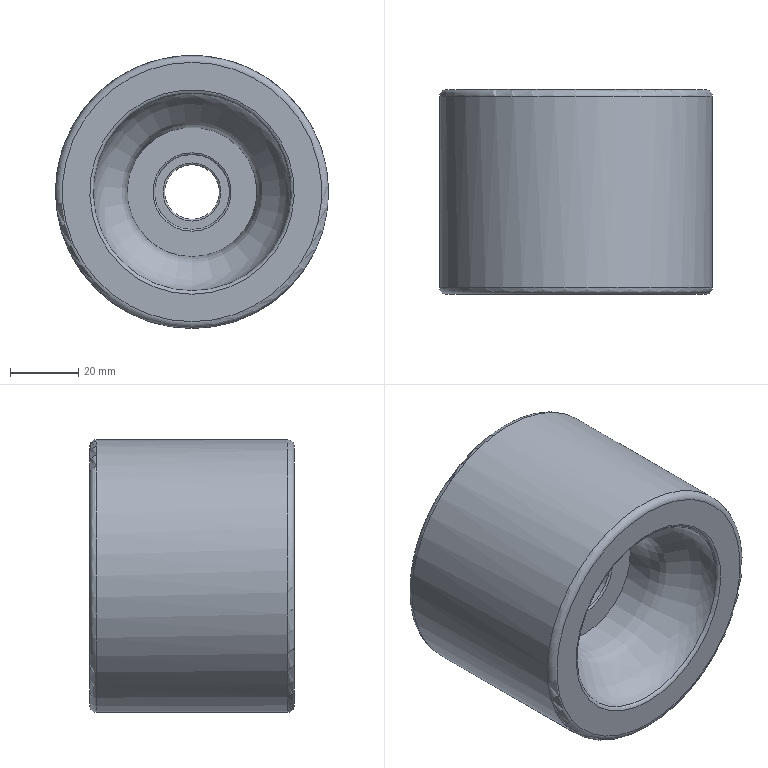Component | NX | WHEEL_2 | 1 solid | 20 faces | volume 227104 mm3 | torus 9 | plane 6 | cylinder 4 | other 1 | commonest cylinder face diameters 22 x2 80 x1 16 x1